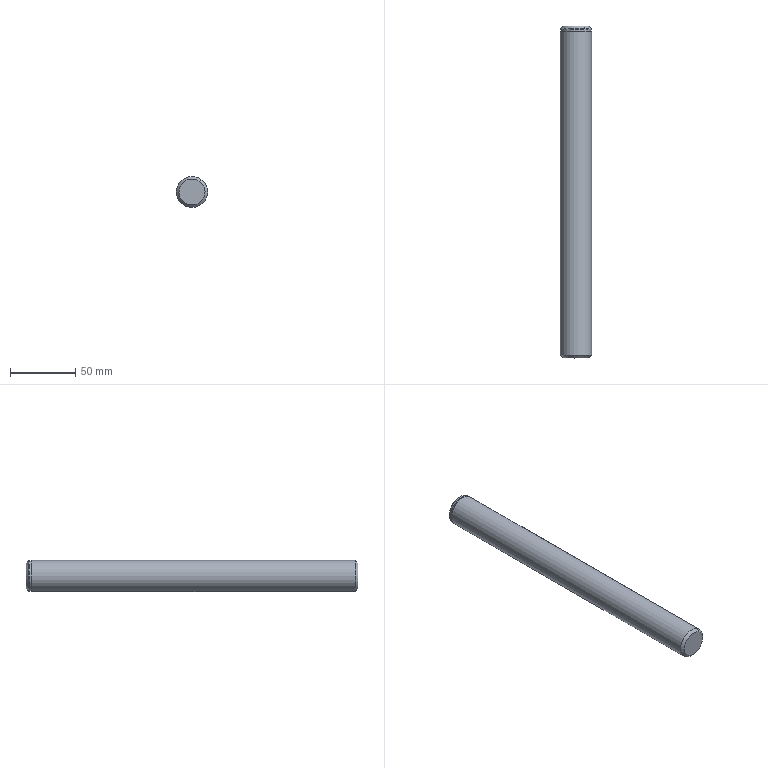Component | SolidWorks | JF21-63.1-17-1-SOLID1-1 | 1 solid | 14 faces | box 24 x 255 x 24 mm | volume 115022 mm3 | cylinder 6 | cone 4 | plane 4 | commonest cylinder face diameters 24 x4 22.9 x2
STEP:
#1=COLOUR_RGB('',0.7922,0.8196,0.9333);
#2=FILL_AREA_STYLE_COLOUR('',#1);
#3=FILL_AREA_STYLE('',(#2));
#4=SURFACE_STYLE_FILL_AREA(#3);
#5=SURFACE_SIDE_STYLE('',(#4));
#6=SURFACE_STYLE_USAGE(.BOTH.,#5);
#7=PRESENTATION_STYLE_ASSIGNMENT((#6));
#8=CARTESIAN_POINT('',(13.607,-32.881,0.3259));
#9=VERTEX_POINT('',#8);
#10=CARTESIAN_POINT('',(13.165,-32.881,-0.3259));
#11=VERTEX_POINT('',#10);
#12=CARTESIAN_POINT('',(13.386,-32.881,-0.));
#13=DIRECTION('',(-0.,-1.,-0.));
#14=DIRECTION('',(0.5609,0.,0.8279));
#15=AXIS2_PLACEMENT_3D('',#12,#13,#14);
#16=CIRCLE('',#15,0.3937);
#17=EDGE_CURVE('',#9,#11,#16,.T.);
#18=ORIENTED_EDGE('',*,*,#17,.F.);
#19=CARTESIAN_POINT('',(13.651,-32.802,0.3911));
#20=VERTEX_POINT('',#19);
#21=CARTESIAN_POINT('',(13.607,-32.881,0.3259));
#22=DIRECTION('',(-0.3966,-0.7071,-0.5854));
#23=VECTOR('',#22,39.37);
#24=LINE('',#21,#23);
#25=EDGE_CURVE('',#20,#9,#24,.T.);
#26=ORIENTED_EDGE('',*,*,#25,.F.);
#27=CARTESIAN_POINT('',(13.121,-32.802,-0.3911));
#28=VERTEX_POINT('',#27);
#29=CARTESIAN_POINT('',(13.386,-32.802,-0.));
#30=DIRECTION('',(0.,1.,0.));
#31=DIRECTION('',(0.5609,0.,0.8279));
#32=AXIS2_PLACEMENT_3D('',#29,#30,#31);
#33=CIRCLE('',#32,0.4724);
#34=EDGE_CURVE('',#28,#20,#33,.T.);
#35=ORIENTED_EDGE('',*,*,#34,.F.);
#36=CARTESIAN_POINT('',(13.165,-32.881,-0.3259));
#37=DIRECTION('',(0.3966,-0.7071,0.5854));
#38=VECTOR('',#37,39.37);
#39=LINE('',#36,#38);
#40=EDGE_CURVE('',#28,#11,#39,.T.);
#41=ORIENTED_EDGE('',*,*,#40,.T.);
#42=EDGE_LOOP('',(#18,#26,#35,#41));
#43=FACE_OUTER_BOUND('',#42,.T.);
#44=CARTESIAN_POINT('',(13.386,-32.881,-0.));
#45=DIRECTION('',(0.,1.,0.));
#46=DIRECTION('',(0.5609,0.,0.8279));
#47=AXIS2_PLACEMENT_3D('',#44,#45,#46);
#48=CONICAL_SURFACE('',#47,0.3937,0.7854);
#49=ADVANCED_FACE('',(#43),#48,.T.);
#50=CARTESIAN_POINT('',(13.165,-22.842,-0.3259));
#51=VERTEX_POINT('',#50);
#52=CARTESIAN_POINT('',(13.607,-22.842,0.3259));
#53=VERTEX_POINT('',#52);
#54=CARTESIAN_POINT('',(13.386,-22.842,-0.));
#55=DIRECTION('',(0.,1.,0.));
#56=DIRECTION('',(-0.5609,0.,-0.8279));
#57=AXIS2_PLACEMENT_3D('',#54,#55,#56);
#58=CIRCLE('',#57,0.3937);
#59=EDGE_CURVE('',#51,#53,#58,.T.);
#60=ORIENTED_EDGE('',*,*,#59,.F.);
#61=CARTESIAN_POINT('',(13.121,-22.92,-0.3911));
#62=VERTEX_POINT('',#61);
#63=CARTESIAN_POINT('',(13.121,-22.92,-0.3911));
#64=DIRECTION('',(-0.3966,-0.7071,-0.5854));
#65=VECTOR('',#64,39.37);
#66=LINE('',#63,#65);
#67=EDGE_CURVE('',#51,#62,#66,.T.);
#68=ORIENTED_EDGE('',*,*,#67,.T.);
#69=CARTESIAN_POINT('',(13.651,-22.92,0.3911));
#70=VERTEX_POINT('',#69);
#71=CARTESIAN_POINT('',(13.386,-22.92,-0.));
#72=DIRECTION('',(-0.,-1.,-0.));
#73=DIRECTION('',(-0.5609,0.,-0.8279));
#74=AXIS2_PLACEMENT_3D('',#71,#72,#73);
#75=CIRCLE('',#74,0.4724);
#76=EDGE_CURVE('',#70,#62,#75,.T.);
#77=ORIENTED_EDGE('',*,*,#76,.F.);
#78=CARTESIAN_POINT('',(13.651,-22.92,0.3911));
#79=DIRECTION('',(0.3966,-0.7071,0.5854));
#80=VECTOR('',#79,39.37);
#81=LINE('',#78,#80);
#82=EDGE_CURVE('',#53,#70,#81,.T.);
#83=ORIENTED_EDGE('',*,*,#82,.F.);
#84=EDGE_LOOP('',(#60,#68,#77,#83));
#85=FACE_OUTER_BOUND('',#84,.T.);
#86=CARTESIAN_POINT('',(13.386,-22.92,-0.));
#87=DIRECTION('',(-0.,-1.,-0.));
#88=DIRECTION('',(-0.5609,0.,-0.8279));
#89=AXIS2_PLACEMENT_3D('',#86,#87,#88);
#90=CONICAL_SURFACE('',#89,0.4724,0.7854);
#91=ADVANCED_FACE('',(#85),#90,.T.);
#92=CARTESIAN_POINT('',(13.651,-23.011,0.3911));
#93=VERTEX_POINT('',#92);
#94=CARTESIAN_POINT('',(13.121,-23.011,-0.3911));
#95=VERTEX_POINT('',#94);
#96=CARTESIAN_POINT('',(13.386,-23.011,-0.));
#97=DIRECTION('',(-0.,-1.,-0.));
#98=DIRECTION('',(0.5609,0.,0.8279));
#99=AXIS2_PLACEMENT_3D('',#96,#97,#98);
#100=CIRCLE('',#99,0.4724);
#101=EDGE_CURVE('',#93,#95,#100,.T.);
#102=ORIENTED_EDGE('',*,*,#101,.T.);
#103=CARTESIAN_POINT('',(13.121,-37.202,-0.3911));
#104=DIRECTION('',(-0.,-1.,-0.));
#105=VECTOR('',#104,39.37);
#106=LINE('',#103,#105);
#107=EDGE_CURVE('',#95,#28,#106,.T.);
#108=ORIENTED_EDGE('',*,*,#107,.T.);
#109=ORIENTED_EDGE('',*,*,#34,.T.);
#110=CARTESIAN_POINT('',(13.651,-37.202,0.3911));
#111=DIRECTION('',(-0.,-1.,-0.));
#112=VECTOR('',#111,39.37);
#113=LINE('',#110,#112);
#114=EDGE_CURVE('',#93,#20,#113,.T.);
#115=ORIENTED_EDGE('',*,*,#114,.F.);
#116=EDGE_LOOP('',(#102,#108,#109,#115));
#117=FACE_OUTER_BOUND('',#116,.T.);
#118=CARTESIAN_POINT('',(13.386,-37.202,-0.));
#119=DIRECTION('',(-0.,-1.,-0.));
#120=DIRECTION('',(-0.5609,0.,-0.8279));
#121=AXIS2_PLACEMENT_3D('',#118,#119,#120);
#122=CYLINDRICAL_SURFACE('',#121,0.4724);
#123=ADVANCED_FACE('',(#117),#122,.T.);
#124=CARTESIAN_POINT('',(13.639,-22.96,0.3732));
#125=VERTEX_POINT('',#124);
#126=CARTESIAN_POINT('',(13.133,-22.96,-0.3732));
#127=VERTEX_POINT('',#126);
#128=CARTESIAN_POINT('',(13.386,-22.96,-0.));
#129=DIRECTION('',(-0.,-1.,-0.));
#130=DIRECTION('',(0.5609,0.,0.8279));
#131=AXIS2_PLACEMENT_3D('',#128,#129,#130);
#132=CIRCLE('',#131,0.4508);
#133=EDGE_CURVE('',#125,#127,#132,.T.);
#134=ORIENTED_EDGE('',*,*,#133,.T.);
#135=CARTESIAN_POINT('',(13.133,-23.011,-0.3732));
#136=VERTEX_POINT('',#135);
#137=CARTESIAN_POINT('',(13.133,-37.202,-0.3732));
#138=DIRECTION('',(-0.,-1.,-0.));
#139=VECTOR('',#138,39.37);
#140=LINE('',#137,#139);
#141=EDGE_CURVE('',#127,#136,#140,.T.);
#142=ORIENTED_EDGE('',*,*,#141,.T.);
#143=CARTESIAN_POINT('',(13.639,-23.011,0.3732));
#144=VERTEX_POINT('',#143);
#145=CARTESIAN_POINT('',(13.386,-23.011,-0.));
#146=DIRECTION('',(-0.,-1.,-0.));
#147=DIRECTION('',(0.5609,0.,0.8279));
#148=AXIS2_PLACEMENT_3D('',#145,#146,#147);
#149=CIRCLE('',#148,0.4508);
#150=EDGE_CURVE('',#144,#136,#149,.T.);
#151=ORIENTED_EDGE('',*,*,#150,.F.);
#152=CARTESIAN_POINT('',(13.639,-37.202,0.3732));
#153=DIRECTION('',(-0.,-1.,-0.));
#154=VECTOR('',#153,39.37);
#155=LINE('',#152,#154);
#156=EDGE_CURVE('',#125,#144,#155,.T.);
#157=ORIENTED_EDGE('',*,*,#156,.F.);
#158=EDGE_LOOP('',(#134,#142,#151,#157));
#159=FACE_OUTER_BOUND('',#158,.T.);
#160=CARTESIAN_POINT('',(13.386,-37.202,-0.));
#161=DIRECTION('',(-0.,-1.,-0.));
#162=DIRECTION('',(-0.5609,0.,-0.8279));
#163=AXIS2_PLACEMENT_3D('',#160,#161,#162);
#164=CYLINDRICAL_SURFACE('',#163,0.4508);
#165=ADVANCED_FACE('',(#159),#164,.T.);
#166=ORIENTED_EDGE('',*,*,#76,.T.);
#167=CARTESIAN_POINT('',(13.121,-22.96,-0.3911));
#168=VERTEX_POINT('',#167);
#169=CARTESIAN_POINT('',(13.121,-37.202,-0.3911));
#170=DIRECTION('',(-0.,-1.,-0.));
#171=VECTOR('',#170,39.37);
#172=LINE('',#169,#171);
#173=EDGE_CURVE('',#62,#168,#172,.T.);
#174=ORIENTED_EDGE('',*,*,#173,.T.);
#175=CARTESIAN_POINT('',(13.651,-22.96,0.3911));
#176=VERTEX_POINT('',#175);
#177=CARTESIAN_POINT('',(13.386,-22.96,-0.));
#178=DIRECTION('',(-0.,-1.,-0.));
#179=DIRECTION('',(0.5609,0.,0.8279));
#180=AXIS2_PLACEMENT_3D('',#177,#178,#179);
#181=CIRCLE('',#180,0.4724);
#182=EDGE_CURVE('',#176,#168,#181,.T.);
#183=ORIENTED_EDGE('',*,*,#182,.F.);
#184=CARTESIAN_POINT('',(13.651,-37.202,0.3911));
#185=DIRECTION('',(-0.,-1.,-0.));
#186=VECTOR('',#185,39.37);
#187=LINE('',#184,#186);
#188=EDGE_CURVE('',#70,#176,#187,.T.);
#189=ORIENTED_EDGE('',*,*,#188,.F.);
#190=EDGE_LOOP('',(#166,#174,#183,#189));
#191=FACE_OUTER_BOUND('',#190,.T.);
#192=CARTESIAN_POINT('',(13.386,-37.202,-0.));
#193=DIRECTION('',(-0.,-1.,-0.));
#194=DIRECTION('',(-0.5609,0.,-0.8279));
#195=AXIS2_PLACEMENT_3D('',#192,#193,#194);
#196=CYLINDRICAL_SURFACE('',#195,0.4724);
#197=ADVANCED_FACE('',(#191),#196,.T.);
#198=CARTESIAN_POINT('',(13.386,-22.842,-0.));
#199=DIRECTION('',(0.,1.,0.));
#200=DIRECTION('',(-0.5609,0.,-0.8279));
#201=AXIS2_PLACEMENT_3D('',#198,#199,#200);
#202=CIRCLE('',#201,0.3937);
#203=EDGE_CURVE('',#53,#51,#202,.T.);
#204=ORIENTED_EDGE('',*,*,#203,.T.);
#205=ORIENTED_EDGE('',*,*,#59,.T.);
#206=EDGE_LOOP('',(#204,#205));
#207=FACE_OUTER_BOUND('',#206,.T.);
#208=CARTESIAN_POINT('',(13.777,-22.842,-0.265));
#209=DIRECTION('',(0.,1.,0.));
#210=DIRECTION('',(0.5609,-0.,0.8279));
#211=AXIS2_PLACEMENT_3D('',#208,#209,#210);
#212=PLANE('',#211);
#213=ADVANCED_FACE('',(#207),#212,.T.);
#214=ORIENTED_EDGE('',*,*,#173,.F.);
#215=CARTESIAN_POINT('',(13.386,-22.92,-0.));
#216=DIRECTION('',(-0.,-1.,-0.));
#217=DIRECTION('',(-0.5609,0.,-0.8279));
#218=AXIS2_PLACEMENT_3D('',#215,#216,#217);
#219=CIRCLE('',#218,0.4724);
#220=EDGE_CURVE('',#62,#70,#219,.T.);
#221=ORIENTED_EDGE('',*,*,#220,.T.);
#222=ORIENTED_EDGE('',*,*,#188,.T.);
#223=CARTESIAN_POINT('',(13.386,-22.96,-0.));
#224=DIRECTION('',(-0.,-1.,-0.));
#225=DIRECTION('',(0.5609,0.,0.8279));
#226=AXIS2_PLACEMENT_3D('',#223,#224,#225);
#227=CIRCLE('',#226,0.4724);
#228=EDGE_CURVE('',#168,#176,#227,.T.);
#229=ORIENTED_EDGE('',*,*,#228,.F.);
#230=EDGE_LOOP('',(#214,#221,#222,#229));
#231=FACE_OUTER_BOUND('',#230,.T.);
#232=CARTESIAN_POINT('',(13.386,-37.202,-0.));
#233=DIRECTION('',(-0.,-1.,-0.));
#234=DIRECTION('',(-0.5609,0.,-0.8279));
#235=AXIS2_PLACEMENT_3D('',#232,#233,#234);
#236=CYLINDRICAL_SURFACE('',#235,0.4724);
#237=ADVANCED_FACE('',(#231),#236,.T.);
#238=ORIENTED_EDGE('',*,*,#182,.T.);
#239=ORIENTED_EDGE('',*,*,#228,.T.);
#240=EDGE_LOOP('',(#238,#239));
#241=FACE_OUTER_BOUND('',#240,.T.);
#242=ORIENTED_EDGE('',*,*,#133,.F.);
#243=CARTESIAN_POINT('',(13.386,-22.96,-0.));
#244=DIRECTION('',(-0.,-1.,-0.));
#245=DIRECTION('',(0.5609,0.,0.8279));
#246=AXIS2_PLACEMENT_3D('',#243,#244,#245);
#247=CIRCLE('',#246,0.4508);
#248=EDGE_CURVE('',#127,#125,#247,.T.);
#249=ORIENTED_EDGE('',*,*,#248,.F.);
#250=EDGE_LOOP('',(#242,#249));
#251=FACE_BOUND('',#250,.T.);
#252=CARTESIAN_POINT('',(13.759,-22.96,-0.2528));
#253=DIRECTION('',(-0.,-1.,-0.));
#254=DIRECTION('',(-0.5609,0.,-0.8279));
#255=AXIS2_PLACEMENT_3D('',#252,#253,#254);
#256=PLANE('',#255);
#257=ADVANCED_FACE('',(#241,#251),#256,.T.);
#258=ORIENTED_EDGE('',*,*,#141,.F.);
#259=ORIENTED_EDGE('',*,*,#248,.T.);
#260=ORIENTED_EDGE('',*,*,#156,.T.);
#261=CARTESIAN_POINT('',(13.386,-23.011,-0.));
#262=DIRECTION('',(-0.,-1.,-0.));
#263=DIRECTION('',(0.5609,0.,0.8279));
#264=AXIS2_PLACEMENT_3D('',#261,#262,#263);
#265=CIRCLE('',#264,0.4508);
#266=EDGE_CURVE('',#136,#144,#265,.T.);
#267=ORIENTED_EDGE('',*,*,#266,.F.);
#268=EDGE_LOOP('',(#258,#259,#260,#267));
#269=FACE_OUTER_BOUND('',#268,.T.);
#270=CARTESIAN_POINT('',(13.386,-37.202,-0.));
#271=DIRECTION('',(-0.,-1.,-0.));
#272=DIRECTION('',(-0.5609,0.,-0.8279));
#273=AXIS2_PLACEMENT_3D('',#270,#271,#272);
#274=CYLINDRICAL_SURFACE('',#273,0.4508);
#275=ADVANCED_FACE('',(#269),#274,.T.);
#276=ORIENTED_EDGE('',*,*,#150,.T.);
#277=ORIENTED_EDGE('',*,*,#266,.T.);
#278=EDGE_LOOP('',(#276,#277));
#279=FACE_BOUND('',#278,.T.);
#280=ORIENTED_EDGE('',*,*,#101,.F.);
#281=CARTESIAN_POINT('',(13.386,-23.011,-0.));
#282=DIRECTION('',(-0.,-1.,-0.));
#283=DIRECTION('',(0.5609,0.,0.8279));
#284=AXIS2_PLACEMENT_3D('',#281,#282,#283);
#285=CIRCLE('',#284,0.4724);
#286=EDGE_CURVE('',#95,#93,#285,.T.);
#287=ORIENTED_EDGE('',*,*,#286,.F.);
#288=EDGE_LOOP('',(#280,#287));
#289=FACE_OUTER_BOUND('',#288,.T.);
#290=CARTESIAN_POINT('',(13.777,-23.011,-0.265));
#291=DIRECTION('',(0.,1.,0.));
#292=DIRECTION('',(0.5609,-0.,0.8279));
#293=AXIS2_PLACEMENT_3D('',#290,#291,#292);
#294=PLANE('',#293);
#295=ADVANCED_FACE('',(#279,#289),#294,.T.);
#296=ORIENTED_EDGE('',*,*,#107,.F.);
#297=ORIENTED_EDGE('',*,*,#286,.T.);
#298=ORIENTED_EDGE('',*,*,#114,.T.);
#299=CARTESIAN_POINT('',(13.386,-32.802,-0.));
#300=DIRECTION('',(0.,1.,0.));
#301=DIRECTION('',(0.5609,0.,0.8279));
#302=AXIS2_PLACEMENT_3D('',#299,#300,#301);
#303=CIRCLE('',#302,0.4724);
#304=EDGE_CURVE('',#20,#28,#303,.T.);
#305=ORIENTED_EDGE('',*,*,#304,.T.);
#306=EDGE_LOOP('',(#296,#297,#298,#305));
#307=FACE_OUTER_BOUND('',#306,.T.);
#308=CARTESIAN_POINT('',(13.386,-37.202,-0.));
#309=DIRECTION('',(-0.,-1.,-0.));
#310=DIRECTION('',(-0.5609,0.,-0.8279));
#311=AXIS2_PLACEMENT_3D('',#308,#309,#310);
#312=CYLINDRICAL_SURFACE('',#311,0.4724);
#313=ADVANCED_FACE('',(#307),#312,.T.);
#314=CARTESIAN_POINT('',(13.386,-32.881,-0.));
#315=DIRECTION('',(-0.,-1.,-0.));
#316=DIRECTION('',(0.5609,0.,0.8279));
#317=AXIS2_PLACEMENT_3D('',#314,#315,#316);
#318=CIRCLE('',#317,0.3937);
#319=EDGE_CURVE('',#11,#9,#318,.T.);
#320=ORIENTED_EDGE('',*,*,#319,.T.);
#321=ORIENTED_EDGE('',*,*,#17,.T.);
#322=EDGE_LOOP('',(#320,#321));
#323=FACE_OUTER_BOUND('',#322,.T.);
#324=CARTESIAN_POINT('',(13.386,-32.881,-0.));
#325=DIRECTION('',(-0.,-1.,-0.));
#326=DIRECTION('',(-0.5609,0.,-0.8279));
#327=AXIS2_PLACEMENT_3D('',#324,#325,#326);
#328=PLANE('',#327);
#329=ADVANCED_FACE('',(#323),#328,.T.);
#330=ORIENTED_EDGE('',*,*,#67,.F.);
#331=ORIENTED_EDGE('',*,*,#203,.F.);
#332=ORIENTED_EDGE('',*,*,#82,.T.);
#333=ORIENTED_EDGE('',*,*,#220,.F.);
#334=EDGE_LOOP('',(#330,#331,#332,#333));
#335=FACE_OUTER_BOUND('',#334,.T.);
#336=CARTESIAN_POINT('',(13.386,-22.92,-0.));
#337=DIRECTION('',(-0.,-1.,-0.));
#338=DIRECTION('',(-0.5609,0.,-0.8279));
#339=AXIS2_PLACEMENT_3D('',#336,#337,#338);
#340=CONICAL_SURFACE('',#339,0.4724,0.7854);
#341=ADVANCED_FACE('',(#335),#340,.T.);
#342=ORIENTED_EDGE('',*,*,#25,.T.);
#343=ORIENTED_EDGE('',*,*,#319,.F.);
#344=ORIENTED_EDGE('',*,*,#40,.F.);
#345=ORIENTED_EDGE('',*,*,#304,.F.);
#346=EDGE_LOOP('',(#342,#343,#344,#345));
#347=FACE_OUTER_BOUND('',#346,.T.);
#348=CARTESIAN_POINT('',(13.386,-32.881,-0.));
#349=DIRECTION('',(0.,1.,0.));
#350=DIRECTION('',(0.5609,0.,0.8279));
#351=AXIS2_PLACEMENT_3D('',#348,#349,#350);
#352=CONICAL_SURFACE('',#351,0.3937,0.7854);
#353=ADVANCED_FACE('',(#347),#352,.T.);
#354=CLOSED_SHELL('',(#49,#91,#123,#165,#197,#213,#237,#257,#275,#295,#313,#329,#341,#353));
#355=MANIFOLD_SOLID_BREP('',#354);
#356=STYLED_ITEM('',(#7),#355);
#357=PRESENTATION_LAYER_ASSIGNMENT('','',(#356));
#358=(LENGTH_UNIT()NAMED_UNIT(*)SI_UNIT($,.METRE.));
#359=LENGTH_MEASURE_WITH_UNIT(LENGTH_MEASURE(0.0254),#358);
#360=DIMENSIONAL_EXPONENTS(1.,0.,0.,0.,0.,0.,0.);
#361=(CONVERSION_BASED_UNIT('',#359)LENGTH_UNIT()NAMED_UNIT(#360));
#362=UNCERTAINTY_MEASURE_WITH_UNIT(LENGTH_MEASURE(0.00001),#361,'','');
#363=(NAMED_UNIT(*)PLANE_ANGLE_UNIT()SI_UNIT($,.RADIAN.));
#364=(NAMED_UNIT(*)SI_UNIT($,.STERADIAN.)SOLID_ANGLE_UNIT());
#365=(GEOMETRIC_REPRESENTATION_CONTEXT(3)GLOBAL_UNCERTAINTY_ASSIGNED_CONTEXT((#362))GLOBAL_UNIT_ASSIGNED_CONTEXT((#361,#363,#364))REPRESENTATION_CONTEXT('',''));
#366=MECHANICAL_DESIGN_GEOMETRIC_PRESENTATION_REPRESENTATION('',(#356),#365);
#367=CARTESIAN_POINT('',(0.,0.,0.));
#368=DIRECTION('',(0.,0.,1.));
#369=DIRECTION('',(1.,0.,0.));
#370=AXIS2_PLACEMENT_3D('',#367,#368,#369);
#371=(LENGTH_UNIT()NAMED_UNIT(*)SI_UNIT($,.METRE.));
#372=LENGTH_MEASURE_WITH_UNIT(LENGTH_MEASURE(0.0254),#371);
#373=DIMENSIONAL_EXPONENTS(1.,0.,0.,0.,0.,0.,0.);
#374=(CONVERSION_BASED_UNIT('',#372)LENGTH_UNIT()NAMED_UNIT(#373));
#375=UNCERTAINTY_MEASURE_WITH_UNIT(LENGTH_MEASURE(0.00001),#374,'','');
#376=(NAMED_UNIT(*)PLANE_ANGLE_UNIT()SI_UNIT($,.RADIAN.));
#377=(NAMED_UNIT(*)SI_UNIT($,.STERADIAN.)SOLID_ANGLE_UNIT());
#378=(GEOMETRIC_REPRESENTATION_CONTEXT(3)GLOBAL_UNCERTAINTY_ASSIGNED_CONTEXT((#375))GLOBAL_UNIT_ASSIGNED_CONTEXT((#374,#376,#377))REPRESENTATION_CONTEXT('',''));
#379=ADVANCED_BREP_SHAPE_REPRESENTATION('',(#355,#370),#378);